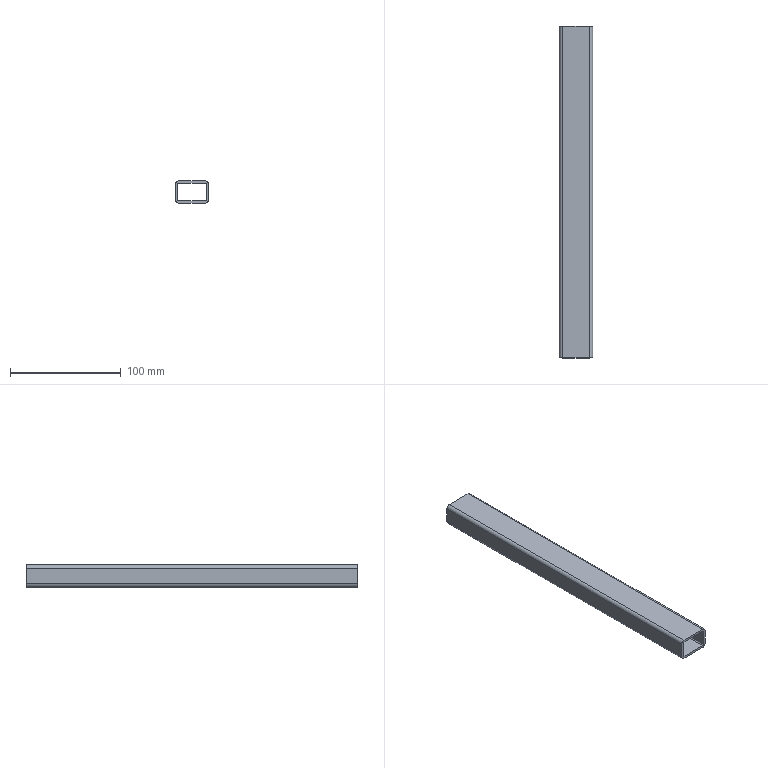Component | SolidWorks | A30x20x2RectangularColdFormedHollowSectionSteel250mm-1 | 1 solid | 18 faces | box 30 x 300 x 20 mm | volume 53140 mm3 | plane 10 | cylinder 8 | commonest cylinder face diameters 6 x4 2 x4
build123d program:
from build123d import *

# Parameters (mm, degrees)
BOSS_EXTRUDE1_DEPTH = 300


with BuildPart() as part:
    # Sketch1 → Boss-Extrude1 (new body)
    with BuildSketch(Plane(origin=(0, 0, 0), x_dir=(0, 0, -1), z_dir=(1, 0, 0))):
        with BuildLine():
            Line((-6.263, 13), (6.263, 13))
            Line((6.263, 13), (7.561, 14.947))
            ThreePointArc((7.561, 14.947), (7.282, 14.987), (7, 15))
            Line((7, 15), (-7, 15))
            ThreePointArc((-7, 15), (-7.282, 14.987), (-7.561, 14.947))
            Line((-7.561, 14.947), (-6.263, 13))
        make_face()
        with BuildLine():
            Line((-10, -11.394), (-8, -8.394))
            Line((-8, -8.394), (-8, 12))
            ThreePointArc((-8, 12), (-7.707, 12.707), (-7, 13))
            Line((-7, 13), (-6.263, 13))
            Line((-6.263, 13), (-7.561, 14.947))
            ThreePointArc((-7.561, 14.947), (-9.311, 13.913), (-10, 12))
            Line((-10, 12), (-10, -11.394))
        make_face()
        with BuildLine():
            Line((8, 12), (8, -8.394))
            Line((8, -8.394), (10, -11.394))
            Line((10, -11.394), (10, 12))
            ThreePointArc((10, 12), (9.311, 13.913), (7.561, 14.947))
            Line((7.561, 14.947), (6.263, 13))
            Line((6.263, 13), (7, 13))
            ThreePointArc((7, 13), (7.707, 12.707), (8, 12))
        make_face()
        with BuildLine():
            Line((7, -13), (-7, -13))
            ThreePointArc((-7, -13), (-7.707, -12.707), (-8, -12))
            Line((-8, -12), (-8, -8.394))
            Line((-8, -8.394), (-10, -11.394))
            Line((-10, -11.394), (-10, -12))
            ThreePointArc((-10, -12), (-9.121, -14.121), (-7, -15))
            Line((-7, -15), (7, -15))
            ThreePointArc((7, -15), (9.121, -14.121), (10, -12))
            Line((10, -12), (10, -11.394))
            Line((10, -11.394), (8, -8.394))
            Line((8, -8.394), (8, -12))
            ThreePointArc((8, -12), (7.707, -12.707), (7, -13))
        make_face()
    extrude(amount=BOSS_EXTRUDE1_DEPTH)


solid = part.part

# Placed as in the assembly
solid = solid.moved(Location((-124.591, -247.9, 400), (0, 0, 90)))
STEP:
#1=COLOUR_RGB('',0.7922,0.8196,0.9333);
#2=FILL_AREA_STYLE_COLOUR('',#1);
#3=FILL_AREA_STYLE('',(#2));
#4=SURFACE_STYLE_FILL_AREA(#3);
#5=SURFACE_SIDE_STYLE('',(#4));
#6=SURFACE_STYLE_USAGE(.BOTH.,#5);
#7=PRESENTATION_STYLE_ASSIGNMENT((#6));
#8=CARTESIAN_POINT('',(-4.433,2.051,16.142));
#9=VERTEX_POINT('',#8);
#10=CARTESIAN_POINT('',(-4.315,2.051,16.024));
#11=VERTEX_POINT('',#10);
#12=CARTESIAN_POINT('',(-4.433,2.051,16.024));
#13=DIRECTION('',(0.,1.,-0.));
#14=DIRECTION('',(0.,0.,-1.));
#15=AXIS2_PLACEMENT_3D('',#12,#13,#14);
#16=CIRCLE('',#15,0.1181);
#17=EDGE_CURVE('',#9,#11,#16,.T.);
#18=ORIENTED_EDGE('',*,*,#17,.F.);
#19=CARTESIAN_POINT('',(-4.433,-9.76,16.142));
#20=VERTEX_POINT('',#19);
#21=CARTESIAN_POINT('',(-4.433,-9.76,16.142));
#22=DIRECTION('',(0.,1.,-0.));
#23=VECTOR('',#22,39.37);
#24=LINE('',#21,#23);
#25=EDGE_CURVE('',#20,#9,#24,.T.);
#26=ORIENTED_EDGE('',*,*,#25,.F.);
#27=CARTESIAN_POINT('',(-4.315,-9.76,16.024));
#28=VERTEX_POINT('',#27);
#29=CARTESIAN_POINT('',(-4.433,-9.76,16.024));
#30=DIRECTION('',(0.,1.,-0.));
#31=DIRECTION('',(0.,0.,-1.));
#32=AXIS2_PLACEMENT_3D('',#29,#30,#31);
#33=CIRCLE('',#32,0.1181);
#34=EDGE_CURVE('',#20,#28,#33,.T.);
#35=ORIENTED_EDGE('',*,*,#34,.T.);
#36=CARTESIAN_POINT('',(-4.315,-9.76,16.024));
#37=DIRECTION('',(0.,1.,-0.));
#38=VECTOR('',#37,39.37);
#39=LINE('',#36,#38);
#40=EDGE_CURVE('',#28,#11,#39,.T.);
#41=ORIENTED_EDGE('',*,*,#40,.T.);
#42=EDGE_LOOP('',(#18,#26,#35,#41));
#43=FACE_OUTER_BOUND('',#42,.T.);
#44=CARTESIAN_POINT('',(-4.433,-9.76,16.024));
#45=DIRECTION('',(0.,1.,-0.));
#46=DIRECTION('',(0.,0.,1.));
#47=AXIS2_PLACEMENT_3D('',#44,#45,#46);
#48=CYLINDRICAL_SURFACE('',#47,0.1181);
#49=ADVANCED_FACE('',(#43),#48,.T.);
#50=CARTESIAN_POINT('',(-5.378,2.051,16.142));
#51=VERTEX_POINT('',#50);
#52=CARTESIAN_POINT('',(-4.905,2.051,16.142));
#53=DIRECTION('',(1.,-0.,-0.));
#54=VECTOR('',#53,39.37);
#55=LINE('',#52,#54);
#56=EDGE_CURVE('',#51,#9,#55,.T.);
#57=ORIENTED_EDGE('',*,*,#56,.F.);
#58=CARTESIAN_POINT('',(-5.378,-9.76,16.142));
#59=VERTEX_POINT('',#58);
#60=CARTESIAN_POINT('',(-5.378,-9.76,16.142));
#61=DIRECTION('',(0.,1.,-0.));
#62=VECTOR('',#61,39.37);
#63=LINE('',#60,#62);
#64=EDGE_CURVE('',#59,#51,#63,.T.);
#65=ORIENTED_EDGE('',*,*,#64,.F.);
#66=CARTESIAN_POINT('',(-4.905,-9.76,16.142));
#67=DIRECTION('',(1.,-0.,-0.));
#68=VECTOR('',#67,39.37);
#69=LINE('',#66,#68);
#70=EDGE_CURVE('',#59,#20,#69,.T.);
#71=ORIENTED_EDGE('',*,*,#70,.T.);
#72=ORIENTED_EDGE('',*,*,#25,.T.);
#73=EDGE_LOOP('',(#57,#65,#71,#72));
#74=FACE_OUTER_BOUND('',#73,.T.);
#75=CARTESIAN_POINT('',(-4.905,-9.76,16.142));
#76=DIRECTION('',(0.,0.,1.));
#77=DIRECTION('',(-0.,-1.,0.));
#78=AXIS2_PLACEMENT_3D('',#75,#76,#77);
#79=PLANE('',#78);
#80=ADVANCED_FACE('',(#74),#79,.T.);
#81=CARTESIAN_POINT('',(-5.496,2.051,16.024));
#82=VERTEX_POINT('',#81);
#83=CARTESIAN_POINT('',(-5.378,2.051,16.024));
#84=DIRECTION('',(0.,1.,-0.));
#85=DIRECTION('',(0.,0.,-1.));
#86=AXIS2_PLACEMENT_3D('',#83,#84,#85);
#87=CIRCLE('',#86,0.1181);
#88=EDGE_CURVE('',#82,#51,#87,.T.);
#89=ORIENTED_EDGE('',*,*,#88,.F.);
#90=CARTESIAN_POINT('',(-5.496,-9.76,16.024));
#91=VERTEX_POINT('',#90);
#92=CARTESIAN_POINT('',(-5.496,-9.76,16.024));
#93=DIRECTION('',(0.,1.,-0.));
#94=VECTOR('',#93,39.37);
#95=LINE('',#92,#94);
#96=EDGE_CURVE('',#91,#82,#95,.T.);
#97=ORIENTED_EDGE('',*,*,#96,.F.);
#98=CARTESIAN_POINT('',(-5.378,-9.76,16.024));
#99=DIRECTION('',(0.,1.,-0.));
#100=DIRECTION('',(0.,0.,-1.));
#101=AXIS2_PLACEMENT_3D('',#98,#99,#100);
#102=CIRCLE('',#101,0.1181);
#103=EDGE_CURVE('',#91,#59,#102,.T.);
#104=ORIENTED_EDGE('',*,*,#103,.T.);
#105=ORIENTED_EDGE('',*,*,#64,.T.);
#106=EDGE_LOOP('',(#89,#97,#104,#105));
#107=FACE_OUTER_BOUND('',#106,.T.);
#108=CARTESIAN_POINT('',(-5.378,-9.76,16.024));
#109=DIRECTION('',(0.,1.,-0.));
#110=DIRECTION('',(0.,0.,1.));
#111=AXIS2_PLACEMENT_3D('',#108,#109,#110);
#112=CYLINDRICAL_SURFACE('',#111,0.1181);
#113=ADVANCED_FACE('',(#107),#112,.T.);
#114=CARTESIAN_POINT('',(-5.496,2.051,15.472));
#115=VERTEX_POINT('',#114);
#116=CARTESIAN_POINT('',(-5.496,2.051,15.748));
#117=DIRECTION('',(-0.,-0.,-1.));
#118=VECTOR('',#117,39.37);
#119=LINE('',#116,#118);
#120=EDGE_CURVE('',#82,#115,#119,.T.);
#121=ORIENTED_EDGE('',*,*,#120,.T.);
#122=CARTESIAN_POINT('',(-5.496,-9.76,15.472));
#123=VERTEX_POINT('',#122);
#124=CARTESIAN_POINT('',(-5.496,-9.76,15.472));
#125=DIRECTION('',(0.,1.,-0.));
#126=VECTOR('',#125,39.37);
#127=LINE('',#124,#126);
#128=EDGE_CURVE('',#123,#115,#127,.T.);
#129=ORIENTED_EDGE('',*,*,#128,.F.);
#130=CARTESIAN_POINT('',(-5.496,-9.76,15.748));
#131=DIRECTION('',(-0.,-0.,-1.));
#132=VECTOR('',#131,39.37);
#133=LINE('',#130,#132);
#134=EDGE_CURVE('',#91,#123,#133,.T.);
#135=ORIENTED_EDGE('',*,*,#134,.F.);
#136=ORIENTED_EDGE('',*,*,#96,.T.);
#137=EDGE_LOOP('',(#121,#129,#135,#136));
#138=FACE_OUTER_BOUND('',#137,.T.);
#139=CARTESIAN_POINT('',(-5.496,-9.76,15.748));
#140=DIRECTION('',(1.,-0.,-0.));
#141=DIRECTION('',(0.,0.,1.));
#142=AXIS2_PLACEMENT_3D('',#139,#140,#141);
#143=PLANE('',#142);
#144=ADVANCED_FACE('',(#138),#143,.F.);
#145=CARTESIAN_POINT('',(-5.378,2.051,15.354));
#146=VERTEX_POINT('',#145);
#147=CARTESIAN_POINT('',(-5.378,2.051,15.472));
#148=DIRECTION('',(-0.,-1.,0.));
#149=DIRECTION('',(0.,0.,-1.));
#150=AXIS2_PLACEMENT_3D('',#147,#148,#149);
#151=CIRCLE('',#150,0.1181);
#152=EDGE_CURVE('',#115,#146,#151,.T.);
#153=ORIENTED_EDGE('',*,*,#152,.T.);
#154=CARTESIAN_POINT('',(-5.378,-9.76,15.354));
#155=VERTEX_POINT('',#154);
#156=CARTESIAN_POINT('',(-5.378,-9.76,15.354));
#157=DIRECTION('',(0.,1.,-0.));
#158=VECTOR('',#157,39.37);
#159=LINE('',#156,#158);
#160=EDGE_CURVE('',#155,#146,#159,.T.);
#161=ORIENTED_EDGE('',*,*,#160,.F.);
#162=CARTESIAN_POINT('',(-5.378,-9.76,15.472));
#163=DIRECTION('',(-0.,-1.,0.));
#164=DIRECTION('',(0.,0.,-1.));
#165=AXIS2_PLACEMENT_3D('',#162,#163,#164);
#166=CIRCLE('',#165,0.1181);
#167=EDGE_CURVE('',#123,#155,#166,.T.);
#168=ORIENTED_EDGE('',*,*,#167,.F.);
#169=ORIENTED_EDGE('',*,*,#128,.T.);
#170=EDGE_LOOP('',(#153,#161,#168,#169));
#171=FACE_OUTER_BOUND('',#170,.T.);
#172=CARTESIAN_POINT('',(-5.378,-9.76,15.472));
#173=DIRECTION('',(0.,1.,-0.));
#174=DIRECTION('',(0.,0.,1.));
#175=AXIS2_PLACEMENT_3D('',#172,#173,#174);
#176=CYLINDRICAL_SURFACE('',#175,0.1181);
#177=ADVANCED_FACE('',(#171),#176,.T.);
#178=CARTESIAN_POINT('',(-4.433,2.051,15.354));
#179=VERTEX_POINT('',#178);
#180=CARTESIAN_POINT('',(-4.905,2.051,15.354));
#181=DIRECTION('',(1.,-0.,-0.));
#182=VECTOR('',#181,39.37);
#183=LINE('',#180,#182);
#184=EDGE_CURVE('',#146,#179,#183,.T.);
#185=ORIENTED_EDGE('',*,*,#184,.T.);
#186=CARTESIAN_POINT('',(-4.433,-9.76,15.354));
#187=VERTEX_POINT('',#186);
#188=CARTESIAN_POINT('',(-4.433,-9.76,15.354));
#189=DIRECTION('',(0.,1.,-0.));
#190=VECTOR('',#189,39.37);
#191=LINE('',#188,#190);
#192=EDGE_CURVE('',#187,#179,#191,.T.);
#193=ORIENTED_EDGE('',*,*,#192,.F.);
#194=CARTESIAN_POINT('',(-4.905,-9.76,15.354));
#195=DIRECTION('',(1.,-0.,-0.));
#196=VECTOR('',#195,39.37);
#197=LINE('',#194,#196);
#198=EDGE_CURVE('',#155,#187,#197,.T.);
#199=ORIENTED_EDGE('',*,*,#198,.F.);
#200=ORIENTED_EDGE('',*,*,#160,.T.);
#201=EDGE_LOOP('',(#185,#193,#199,#200));
#202=FACE_OUTER_BOUND('',#201,.T.);
#203=CARTESIAN_POINT('',(-4.905,-9.76,15.354));
#204=DIRECTION('',(0.,0.,1.));
#205=DIRECTION('',(-0.,-1.,0.));
#206=AXIS2_PLACEMENT_3D('',#203,#204,#205);
#207=PLANE('',#206);
#208=ADVANCED_FACE('',(#202),#207,.F.);
#209=CARTESIAN_POINT('',(-4.315,2.051,15.472));
#210=VERTEX_POINT('',#209);
#211=CARTESIAN_POINT('',(-4.433,2.051,15.472));
#212=DIRECTION('',(0.,1.,-0.));
#213=DIRECTION('',(0.,0.,-1.));
#214=AXIS2_PLACEMENT_3D('',#211,#212,#213);
#215=CIRCLE('',#214,0.1181);
#216=EDGE_CURVE('',#210,#179,#215,.T.);
#217=ORIENTED_EDGE('',*,*,#216,.F.);
#218=CARTESIAN_POINT('',(-4.315,-9.76,15.472));
#219=VERTEX_POINT('',#218);
#220=CARTESIAN_POINT('',(-4.315,-9.76,15.472));
#221=DIRECTION('',(0.,1.,-0.));
#222=VECTOR('',#221,39.37);
#223=LINE('',#220,#222);
#224=EDGE_CURVE('',#219,#210,#223,.T.);
#225=ORIENTED_EDGE('',*,*,#224,.F.);
#226=CARTESIAN_POINT('',(-4.433,-9.76,15.472));
#227=DIRECTION('',(0.,1.,-0.));
#228=DIRECTION('',(0.,0.,-1.));
#229=AXIS2_PLACEMENT_3D('',#226,#227,#228);
#230=CIRCLE('',#229,0.1181);
#231=EDGE_CURVE('',#219,#187,#230,.T.);
#232=ORIENTED_EDGE('',*,*,#231,.T.);
#233=ORIENTED_EDGE('',*,*,#192,.T.);
#234=EDGE_LOOP('',(#217,#225,#232,#233));
#235=FACE_OUTER_BOUND('',#234,.T.);
#236=CARTESIAN_POINT('',(-4.433,-9.76,15.472));
#237=DIRECTION('',(0.,1.,-0.));
#238=DIRECTION('',(0.,0.,1.));
#239=AXIS2_PLACEMENT_3D('',#236,#237,#238);
#240=CYLINDRICAL_SURFACE('',#239,0.1181);
#241=ADVANCED_FACE('',(#235),#240,.T.);
#242=CARTESIAN_POINT('',(-5.417,2.051,16.024));
#243=VERTEX_POINT('',#242);
#244=CARTESIAN_POINT('',(-5.378,2.051,16.063));
#245=VERTEX_POINT('',#244);
#246=CARTESIAN_POINT('',(-5.378,2.051,16.024));
#247=DIRECTION('',(0.,1.,-0.));
#248=DIRECTION('',(0.,0.,-1.));
#249=AXIS2_PLACEMENT_3D('',#246,#247,#248);
#250=CIRCLE('',#249,0.03937);
#251=EDGE_CURVE('',#243,#245,#250,.T.);
#252=ORIENTED_EDGE('',*,*,#251,.T.);
#253=CARTESIAN_POINT('',(-5.378,-9.76,16.063));
#254=VERTEX_POINT('',#253);
#255=CARTESIAN_POINT('',(-5.378,-9.76,16.063));
#256=DIRECTION('',(0.,1.,-0.));
#257=VECTOR('',#256,39.37);
#258=LINE('',#255,#257);
#259=EDGE_CURVE('',#254,#245,#258,.T.);
#260=ORIENTED_EDGE('',*,*,#259,.F.);
#261=CARTESIAN_POINT('',(-5.417,-9.76,16.024));
#262=VERTEX_POINT('',#261);
#263=CARTESIAN_POINT('',(-5.378,-9.76,16.024));
#264=DIRECTION('',(0.,1.,-0.));
#265=DIRECTION('',(0.,0.,-1.));
#266=AXIS2_PLACEMENT_3D('',#263,#264,#265);
#267=CIRCLE('',#266,0.03937);
#268=EDGE_CURVE('',#262,#254,#267,.T.);
#269=ORIENTED_EDGE('',*,*,#268,.F.);
#270=CARTESIAN_POINT('',(-5.417,-9.76,16.024));
#271=DIRECTION('',(0.,1.,-0.));
#272=VECTOR('',#271,39.37);
#273=LINE('',#270,#272);
#274=EDGE_CURVE('',#262,#243,#273,.T.);
#275=ORIENTED_EDGE('',*,*,#274,.T.);
#276=EDGE_LOOP('',(#252,#260,#269,#275));
#277=FACE_OUTER_BOUND('',#276,.T.);
#278=CARTESIAN_POINT('',(-5.378,-9.76,16.024));
#279=DIRECTION('',(0.,1.,-0.));
#280=DIRECTION('',(0.,0.,1.));
#281=AXIS2_PLACEMENT_3D('',#278,#279,#280);
#282=CYLINDRICAL_SURFACE('',#281,0.03937);
#283=ADVANCED_FACE('',(#277),#282,.F.);
#284=CARTESIAN_POINT('',(-4.433,2.051,16.063));
#285=VERTEX_POINT('',#284);
#286=CARTESIAN_POINT('',(-4.905,2.051,16.063));
#287=DIRECTION('',(1.,-0.,-0.));
#288=VECTOR('',#287,39.37);
#289=LINE('',#286,#288);
#290=EDGE_CURVE('',#245,#285,#289,.T.);
#291=ORIENTED_EDGE('',*,*,#290,.T.);
#292=CARTESIAN_POINT('',(-4.433,-9.76,16.063));
#293=VERTEX_POINT('',#292);
#294=CARTESIAN_POINT('',(-4.433,-9.76,16.063));
#295=DIRECTION('',(0.,1.,-0.));
#296=VECTOR('',#295,39.37);
#297=LINE('',#294,#296);
#298=EDGE_CURVE('',#293,#285,#297,.T.);
#299=ORIENTED_EDGE('',*,*,#298,.F.);
#300=CARTESIAN_POINT('',(-4.905,-9.76,16.063));
#301=DIRECTION('',(1.,-0.,-0.));
#302=VECTOR('',#301,39.37);
#303=LINE('',#300,#302);
#304=EDGE_CURVE('',#254,#293,#303,.T.);
#305=ORIENTED_EDGE('',*,*,#304,.F.);
#306=ORIENTED_EDGE('',*,*,#259,.T.);
#307=EDGE_LOOP('',(#291,#299,#305,#306));
#308=FACE_OUTER_BOUND('',#307,.T.);
#309=CARTESIAN_POINT('',(-4.905,-9.76,16.063));
#310=DIRECTION('',(0.,0.,1.));
#311=DIRECTION('',(-0.,-1.,0.));
#312=AXIS2_PLACEMENT_3D('',#309,#310,#311);
#313=PLANE('',#312);
#314=ADVANCED_FACE('',(#308),#313,.F.);
#315=CARTESIAN_POINT('',(-4.393,2.051,16.024));
#316=VERTEX_POINT('',#315);
#317=CARTESIAN_POINT('',(-4.433,2.051,16.024));
#318=DIRECTION('',(0.,1.,-0.));
#319=DIRECTION('',(0.,0.,-1.));
#320=AXIS2_PLACEMENT_3D('',#317,#318,#319);
#321=CIRCLE('',#320,0.03937);
#322=EDGE_CURVE('',#285,#316,#321,.T.);
#323=ORIENTED_EDGE('',*,*,#322,.T.);
#324=CARTESIAN_POINT('',(-4.393,-9.76,16.024));
#325=VERTEX_POINT('',#324);
#326=CARTESIAN_POINT('',(-4.393,-9.76,16.024));
#327=DIRECTION('',(0.,1.,-0.));
#328=VECTOR('',#327,39.37);
#329=LINE('',#326,#328);
#330=EDGE_CURVE('',#325,#316,#329,.T.);
#331=ORIENTED_EDGE('',*,*,#330,.F.);
#332=CARTESIAN_POINT('',(-4.433,-9.76,16.024));
#333=DIRECTION('',(0.,1.,-0.));
#334=DIRECTION('',(0.,0.,-1.));
#335=AXIS2_PLACEMENT_3D('',#332,#333,#334);
#336=CIRCLE('',#335,0.03937);
#337=EDGE_CURVE('',#293,#325,#336,.T.);
#338=ORIENTED_EDGE('',*,*,#337,.F.);
#339=ORIENTED_EDGE('',*,*,#298,.T.);
#340=EDGE_LOOP('',(#323,#331,#338,#339));
#341=FACE_OUTER_BOUND('',#340,.T.);
#342=CARTESIAN_POINT('',(-4.433,-9.76,16.024));
#343=DIRECTION('',(0.,1.,-0.));
#344=DIRECTION('',(0.,0.,1.));
#345=AXIS2_PLACEMENT_3D('',#342,#343,#344);
#346=CYLINDRICAL_SURFACE('',#345,0.03937);
#347=ADVANCED_FACE('',(#341),#346,.F.);
#348=CARTESIAN_POINT('',(-4.393,2.051,15.472));
#349=VERTEX_POINT('',#348);
#350=CARTESIAN_POINT('',(-4.393,2.051,15.748));
#351=DIRECTION('',(-0.,-0.,-1.));
#352=VECTOR('',#351,39.37);
#353=LINE('',#350,#352);
#354=EDGE_CURVE('',#316,#349,#353,.T.);
#355=ORIENTED_EDGE('',*,*,#354,.T.);
#356=CARTESIAN_POINT('',(-4.393,-9.76,15.472));
#357=VERTEX_POINT('',#356);
#358=CARTESIAN_POINT('',(-4.393,-9.76,15.472));
#359=DIRECTION('',(0.,1.,-0.));
#360=VECTOR('',#359,39.37);
#361=LINE('',#358,#360);
#362=EDGE_CURVE('',#357,#349,#361,.T.);
#363=ORIENTED_EDGE('',*,*,#362,.F.);
#364=CARTESIAN_POINT('',(-4.393,-9.76,15.748));
#365=DIRECTION('',(-0.,-0.,-1.));
#366=VECTOR('',#365,39.37);
#367=LINE('',#364,#366);
#368=EDGE_CURVE('',#325,#357,#367,.T.);
#369=ORIENTED_EDGE('',*,*,#368,.F.);
#370=ORIENTED_EDGE('',*,*,#330,.T.);
#371=EDGE_LOOP('',(#355,#363,#369,#370));
#372=FACE_OUTER_BOUND('',#371,.T.);
#373=CARTESIAN_POINT('',(-4.393,-9.76,15.748));
#374=DIRECTION('',(1.,-0.,-0.));
#375=DIRECTION('',(0.,0.,1.));
#376=AXIS2_PLACEMENT_3D('',#373,#374,#375);
#377=PLANE('',#376);
#378=ADVANCED_FACE('',(#372),#377,.F.);
#379=CARTESIAN_POINT('',(-4.433,2.051,15.433));
#380=VERTEX_POINT('',#379);
#381=CARTESIAN_POINT('',(-4.433,2.051,15.472));
#382=DIRECTION('',(0.,1.,-0.));
#383=DIRECTION('',(0.,0.,-1.));
#384=AXIS2_PLACEMENT_3D('',#381,#382,#383);
#385=CIRCLE('',#384,0.03937);
#386=EDGE_CURVE('',#349,#380,#385,.T.);
#387=ORIENTED_EDGE('',*,*,#386,.T.);
#388=CARTESIAN_POINT('',(-4.433,-9.76,15.433));
#389=VERTEX_POINT('',#388);
#390=CARTESIAN_POINT('',(-4.433,-9.76,15.433));
#391=DIRECTION('',(0.,1.,-0.));
#392=VECTOR('',#391,39.37);
#393=LINE('',#390,#392);
#394=EDGE_CURVE('',#389,#380,#393,.T.);
#395=ORIENTED_EDGE('',*,*,#394,.F.);
#396=CARTESIAN_POINT('',(-4.433,-9.76,15.472));
#397=DIRECTION('',(0.,1.,-0.));
#398=DIRECTION('',(0.,0.,-1.));
#399=AXIS2_PLACEMENT_3D('',#396,#397,#398);
#400=CIRCLE('',#399,0.03937);
#401=EDGE_CURVE('',#357,#389,#400,.T.);
#402=ORIENTED_EDGE('',*,*,#401,.F.);
#403=ORIENTED_EDGE('',*,*,#362,.T.);
#404=EDGE_LOOP('',(#387,#395,#402,#403));
#405=FACE_OUTER_BOUND('',#404,.T.);
#406=CARTESIAN_POINT('',(-4.433,-9.76,15.472));
#407=DIRECTION('',(0.,1.,-0.));
#408=DIRECTION('',(0.,0.,1.));
#409=AXIS2_PLACEMENT_3D('',#406,#407,#408);
#410=CYLINDRICAL_SURFACE('',#409,0.03937);
#411=ADVANCED_FACE('',(#405),#410,.F.);
#412=CARTESIAN_POINT('',(-5.378,2.051,15.433));
#413=VERTEX_POINT('',#412);
#414=CARTESIAN_POINT('',(-4.905,2.051,15.433));
#415=DIRECTION('',(1.,-0.,-0.));
#416=VECTOR('',#415,39.37);
#417=LINE('',#414,#416);
#418=EDGE_CURVE('',#413,#380,#417,.T.);
#419=ORIENTED_EDGE('',*,*,#418,.F.);
#420=CARTESIAN_POINT('',(-5.378,-9.76,15.433));
#421=VERTEX_POINT('',#420);
#422=CARTESIAN_POINT('',(-5.378,-9.76,15.433));
#423=DIRECTION('',(0.,1.,-0.));
#424=VECTOR('',#423,39.37);
#425=LINE('',#422,#424);
#426=EDGE_CURVE('',#421,#413,#425,.T.);
#427=ORIENTED_EDGE('',*,*,#426,.F.);
#428=CARTESIAN_POINT('',(-4.905,-9.76,15.433));
#429=DIRECTION('',(1.,-0.,-0.));
#430=VECTOR('',#429,39.37);
#431=LINE('',#428,#430);
#432=EDGE_CURVE('',#421,#389,#431,.T.);
#433=ORIENTED_EDGE('',*,*,#432,.T.);
#434=ORIENTED_EDGE('',*,*,#394,.T.);
#435=EDGE_LOOP('',(#419,#427,#433,#434));
#436=FACE_OUTER_BOUND('',#435,.T.);
#437=CARTESIAN_POINT('',(-4.905,-9.76,15.433));
#438=DIRECTION('',(0.,0.,1.));
#439=DIRECTION('',(-0.,-1.,0.));
#440=AXIS2_PLACEMENT_3D('',#437,#438,#439);
#441=PLANE('',#440);
#442=ADVANCED_FACE('',(#436),#441,.T.);
#443=CARTESIAN_POINT('',(-5.417,2.051,15.472));
#444=VERTEX_POINT('',#443);
#445=CARTESIAN_POINT('',(-5.378,2.051,15.472));
#446=DIRECTION('',(-0.,-1.,0.));
#447=DIRECTION('',(0.,0.,-1.));
#448=AXIS2_PLACEMENT_3D('',#445,#446,#447);
#449=CIRCLE('',#448,0.03937);
#450=EDGE_CURVE('',#444,#413,#449,.T.);
#451=ORIENTED_EDGE('',*,*,#450,.F.);
#452=CARTESIAN_POINT('',(-5.417,-9.76,15.472));
#453=VERTEX_POINT('',#452);
#454=CARTESIAN_POINT('',(-5.417,-9.76,15.472));
#455=DIRECTION('',(0.,1.,-0.));
#456=VECTOR('',#455,39.37);
#457=LINE('',#454,#456);
#458=EDGE_CURVE('',#453,#444,#457,.T.);
#459=ORIENTED_EDGE('',*,*,#458,.F.);
#460=CARTESIAN_POINT('',(-5.378,-9.76,15.472));
#461=DIRECTION('',(-0.,-1.,0.));
#462=DIRECTION('',(0.,0.,-1.));
#463=AXIS2_PLACEMENT_3D('',#460,#461,#462);
#464=CIRCLE('',#463,0.03937);
#465=EDGE_CURVE('',#453,#421,#464,.T.);
#466=ORIENTED_EDGE('',*,*,#465,.T.);
#467=ORIENTED_EDGE('',*,*,#426,.T.);
#468=EDGE_LOOP('',(#451,#459,#466,#467));
#469=FACE_OUTER_BOUND('',#468,.T.);
#470=CARTESIAN_POINT('',(-5.378,-9.76,15.472));
#471=DIRECTION('',(0.,1.,-0.));
#472=DIRECTION('',(0.,0.,1.));
#473=AXIS2_PLACEMENT_3D('',#470,#471,#472);
#474=CYLINDRICAL_SURFACE('',#473,0.03937);
#475=ADVANCED_FACE('',(#469),#474,.F.);
#476=CARTESIAN_POINT('',(-5.417,2.051,15.748));
#477=DIRECTION('',(-0.,-0.,-1.));
#478=VECTOR('',#477,39.37);
#479=LINE('',#476,#478);
#480=EDGE_CURVE('',#243,#444,#479,.T.);
#481=ORIENTED_EDGE('',*,*,#480,.F.);
#482=ORIENTED_EDGE('',*,*,#274,.F.);
#483=CARTESIAN_POINT('',(-5.417,-9.76,15.748));
#484=DIRECTION('',(-0.,-0.,-1.));
#485=VECTOR('',#484,39.37);
#486=LINE('',#483,#485);
#487=EDGE_CURVE('',#262,#453,#486,.T.);
#488=ORIENTED_EDGE('',*,*,#487,.T.);
#489=ORIENTED_EDGE('',*,*,#458,.T.);
#490=EDGE_LOOP('',(#481,#482,#488,#489));
#491=FACE_OUTER_BOUND('',#490,.T.);
#492=CARTESIAN_POINT('',(-5.417,-9.76,15.748));
#493=DIRECTION('',(1.,-0.,-0.));
#494=DIRECTION('',(0.,0.,1.));
#495=AXIS2_PLACEMENT_3D('',#492,#493,#494);
#496=PLANE('',#495);
#497=ADVANCED_FACE('',(#491),#496,.T.);
#498=CARTESIAN_POINT('',(-4.315,2.051,15.748));
#499=DIRECTION('',(-0.,-0.,-1.));
#500=VECTOR('',#499,39.37);
#501=LINE('',#498,#500);
#502=EDGE_CURVE('',#11,#210,#501,.T.);
#503=ORIENTED_EDGE('',*,*,#502,.F.);
#504=ORIENTED_EDGE('',*,*,#40,.F.);
#505=CARTESIAN_POINT('',(-4.315,-9.76,15.748));
#506=DIRECTION('',(-0.,-0.,-1.));
#507=VECTOR('',#506,39.37);
#508=LINE('',#505,#507);
#509=EDGE_CURVE('',#28,#219,#508,.T.);
#510=ORIENTED_EDGE('',*,*,#509,.T.);
#511=ORIENTED_EDGE('',*,*,#224,.T.);
#512=EDGE_LOOP('',(#503,#504,#510,#511));
#513=FACE_OUTER_BOUND('',#512,.T.);
#514=CARTESIAN_POINT('',(-4.315,-9.76,15.748));
#515=DIRECTION('',(1.,-0.,-0.));
#516=DIRECTION('',(0.,0.,1.));
#517=AXIS2_PLACEMENT_3D('',#514,#515,#516);
#518=PLANE('',#517);
#519=ADVANCED_FACE('',(#513),#518,.T.);
#520=ORIENTED_EDGE('',*,*,#268,.T.);
#521=ORIENTED_EDGE('',*,*,#304,.T.);
#522=ORIENTED_EDGE('',*,*,#337,.T.);
#523=ORIENTED_EDGE('',*,*,#368,.T.);
#524=ORIENTED_EDGE('',*,*,#401,.T.);
#525=ORIENTED_EDGE('',*,*,#432,.F.);
#526=ORIENTED_EDGE('',*,*,#465,.F.);
#527=ORIENTED_EDGE('',*,*,#487,.F.);
#528=EDGE_LOOP('',(#520,#521,#522,#523,#524,#525,#526,#527));
#529=FACE_BOUND('',#528,.T.);
#530=ORIENTED_EDGE('',*,*,#34,.F.);
#531=ORIENTED_EDGE('',*,*,#70,.F.);
#532=ORIENTED_EDGE('',*,*,#103,.F.);
#533=ORIENTED_EDGE('',*,*,#134,.T.);
#534=ORIENTED_EDGE('',*,*,#167,.T.);
#535=ORIENTED_EDGE('',*,*,#198,.T.);
#536=ORIENTED_EDGE('',*,*,#231,.F.);
#537=ORIENTED_EDGE('',*,*,#509,.F.);
#538=EDGE_LOOP('',(#530,#531,#532,#533,#534,#535,#536,#537));
#539=FACE_OUTER_BOUND('',#538,.T.);
#540=CARTESIAN_POINT('',(-4.905,-9.76,15.748));
#541=DIRECTION('',(-0.,-1.,0.));
#542=DIRECTION('',(-0.,-0.,-1.));
#543=AXIS2_PLACEMENT_3D('',#540,#541,#542);
#544=PLANE('',#543);
#545=ADVANCED_FACE('',(#529,#539),#544,.T.);
#546=ORIENTED_EDGE('',*,*,#251,.F.);
#547=ORIENTED_EDGE('',*,*,#480,.T.);
#548=ORIENTED_EDGE('',*,*,#450,.T.);
#549=ORIENTED_EDGE('',*,*,#418,.T.);
#550=ORIENTED_EDGE('',*,*,#386,.F.);
#551=ORIENTED_EDGE('',*,*,#354,.F.);
#552=ORIENTED_EDGE('',*,*,#322,.F.);
#553=ORIENTED_EDGE('',*,*,#290,.F.);
#554=EDGE_LOOP('',(#546,#547,#548,#549,#550,#551,#552,#553));
#555=FACE_BOUND('',#554,.T.);
#556=ORIENTED_EDGE('',*,*,#17,.T.);
#557=ORIENTED_EDGE('',*,*,#502,.T.);
#558=ORIENTED_EDGE('',*,*,#216,.T.);
#559=ORIENTED_EDGE('',*,*,#184,.F.);
#560=ORIENTED_EDGE('',*,*,#152,.F.);
#561=ORIENTED_EDGE('',*,*,#120,.F.);
#562=ORIENTED_EDGE('',*,*,#88,.T.);
#563=ORIENTED_EDGE('',*,*,#56,.T.);
#564=EDGE_LOOP('',(#556,#557,#558,#559,#560,#561,#562,#563));
#565=FACE_OUTER_BOUND('',#564,.T.);
#566=CARTESIAN_POINT('',(-4.905,2.051,15.748));
#567=DIRECTION('',(-0.,-1.,0.));
#568=DIRECTION('',(-0.,-0.,-1.));
#569=AXIS2_PLACEMENT_3D('',#566,#567,#568);
#570=PLANE('',#569);
#571=ADVANCED_FACE('',(#555,#565),#570,.F.);
#572=CLOSED_SHELL('',(#49,#80,#113,#144,#177,#208,#241,#283,#314,#347,#378,#411,#442,#475,#497,#519,#545,#571));
#573=MANIFOLD_SOLID_BREP('',#572);
#574=STYLED_ITEM('',(#7),#573);
#575=(LENGTH_UNIT()NAMED_UNIT(*)SI_UNIT($,.METRE.));
#576=LENGTH_MEASURE_WITH_UNIT(LENGTH_MEASURE(0.0254),#575);
#577=DIMENSIONAL_EXPONENTS(1.,0.,0.,0.,0.,0.,0.);
#578=(CONVERSION_BASED_UNIT('',#576)LENGTH_UNIT()NAMED_UNIT(#577));
#579=UNCERTAINTY_MEASURE_WITH_UNIT(LENGTH_MEASURE(0.00001),#578,'','');
#580=(NAMED_UNIT(*)PLANE_ANGLE_UNIT()SI_UNIT($,.RADIAN.));
#581=(NAMED_UNIT(*)SI_UNIT($,.STERADIAN.)SOLID_ANGLE_UNIT());
#582=(GEOMETRIC_REPRESENTATION_CONTEXT(3)GLOBAL_UNCERTAINTY_ASSIGNED_CONTEXT((#579))GLOBAL_UNIT_ASSIGNED_CONTEXT((#578,#580,#581))REPRESENTATION_CONTEXT('',''));
#583=MECHANICAL_DESIGN_GEOMETRIC_PRESENTATION_REPRESENTATION('',(#574),#582);
#584=CARTESIAN_POINT('',(0.,0.,0.));
#585=DIRECTION('',(0.,0.,1.));
#586=DIRECTION('',(1.,0.,0.));
#587=AXIS2_PLACEMENT_3D('',#584,#585,#586);
#588=(LENGTH_UNIT()NAMED_UNIT(*)SI_UNIT($,.METRE.));
#589=LENGTH_MEASURE_WITH_UNIT(LENGTH_MEASURE(0.0254),#588);
#590=DIMENSIONAL_EXPONENTS(1.,0.,0.,0.,0.,0.,0.);
#591=(CONVERSION_BASED_UNIT('',#589)LENGTH_UNIT()NAMED_UNIT(#590));
#592=UNCERTAINTY_MEASURE_WITH_UNIT(LENGTH_MEASURE(0.00001),#591,'','');
#593=(NAMED_UNIT(*)PLANE_ANGLE_UNIT()SI_UNIT($,.RADIAN.));
#594=(NAMED_UNIT(*)SI_UNIT($,.STERADIAN.)SOLID_ANGLE_UNIT());
#595=(GEOMETRIC_REPRESENTATION_CONTEXT(3)GLOBAL_UNCERTAINTY_ASSIGNED_CONTEXT((#592))GLOBAL_UNIT_ASSIGNED_CONTEXT((#591,#593,#594))REPRESENTATION_CONTEXT('',''));
#596=ADVANCED_BREP_SHAPE_REPRESENTATION('',(#573,#587),#595);
#597=PRESENTATION_LAYER_ASSIGNMENT('','',(#574));